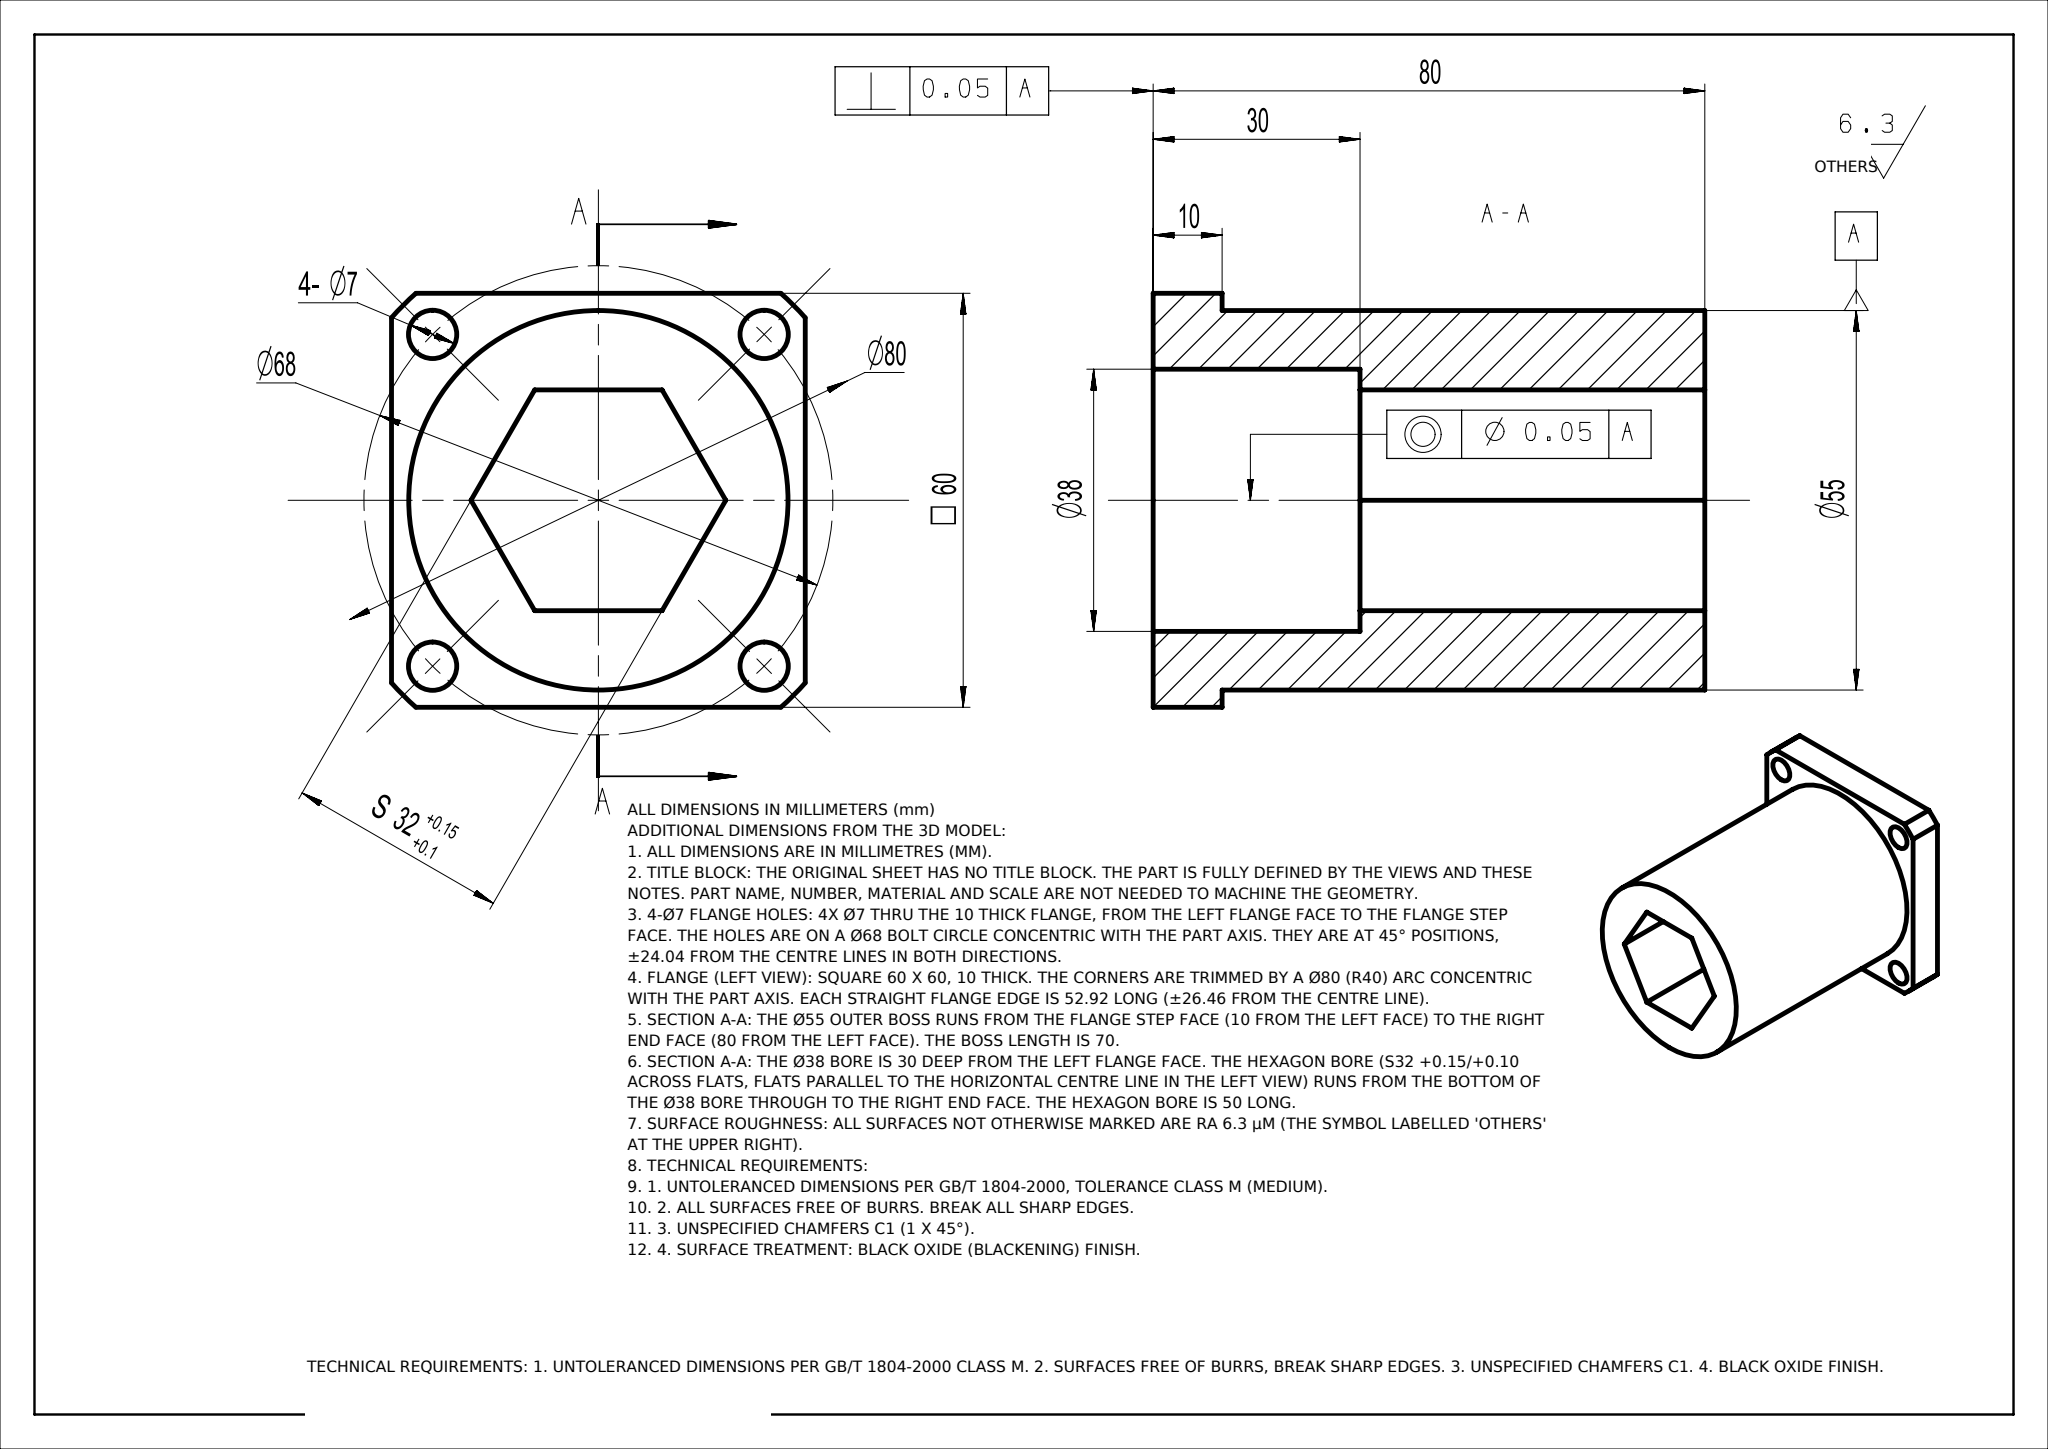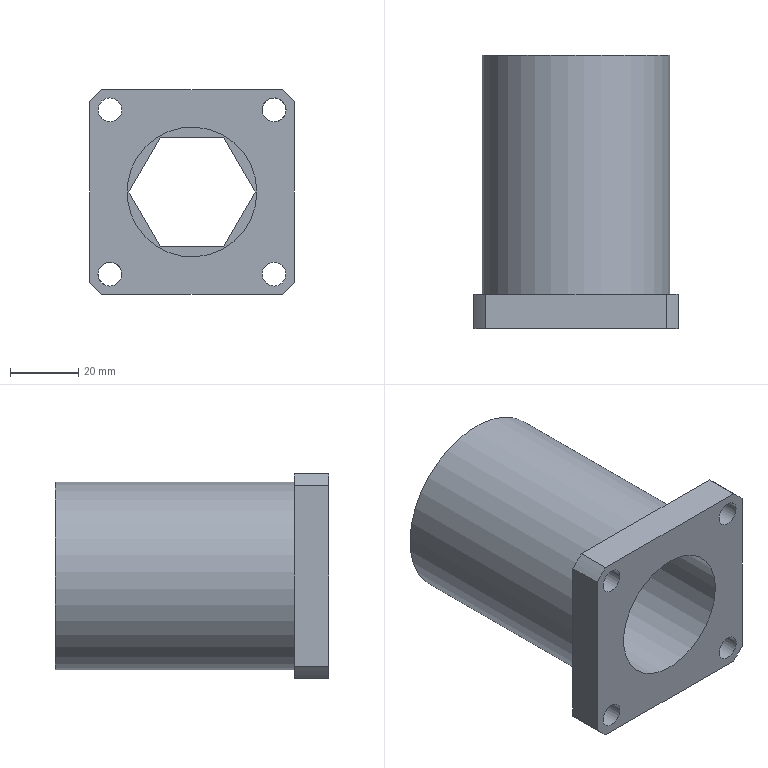Part | NX | mm | 1 solid | 24 faces | box 60 x 80 x 60 mm | volume 122164 mm3 | plane 14 | cylinder 10 | commonest cylinder face diameters 80 x4 7 x4 55 x1 38 x1
STEP:
#1=CARTESIAN_POINT('',(0.,0.,0.));
#2=DIRECTION('',(0.,0.,1.));
#3=DIRECTION('',(1.,0.,0.));
#4=AXIS2_PLACEMENT_3D('',#1,#2,#3);
#5=(LENGTH_UNIT()NAMED_UNIT(*)SI_UNIT(.MILLI.,.METRE.));
#6=UNCERTAINTY_MEASURE_WITH_UNIT(LENGTH_MEASURE(0.00002),#5,'','');
#7=(NAMED_UNIT(*)PLANE_ANGLE_UNIT()SI_UNIT($,.RADIAN.));
#8=PLANE_ANGLE_MEASURE_WITH_UNIT(PLANE_ANGLE_MEASURE(0.01745),#7);
#9=DIMENSIONAL_EXPONENTS(0.,0.,0.,0.,0.,0.,0.);
#10=(CONVERSION_BASED_UNIT('',#8)NAMED_UNIT(#9)PLANE_ANGLE_UNIT());
#11=(NAMED_UNIT(*)SI_UNIT($,.STERADIAN.)SOLID_ANGLE_UNIT());
#12=(GEOMETRIC_REPRESENTATION_CONTEXT(3)GLOBAL_UNCERTAINTY_ASSIGNED_CONTEXT((#6))GLOBAL_UNIT_ASSIGNED_CONTEXT((#5,#10,#11))REPRESENTATION_CONTEXT('',''));
#13=SHAPE_REPRESENTATION('',(#4),#12);
#14=CARTESIAN_POINT('',(-26.458,10.,30.));
#15=VERTEX_POINT('',#14);
#16=CARTESIAN_POINT('',(-30.,10.,26.458));
#17=VERTEX_POINT('',#16);
#18=CARTESIAN_POINT('',(0.,10.,0.));
#19=DIRECTION('',(0.,-1.,0.));
#20=DIRECTION('',(0.,-0.,-1.));
#21=AXIS2_PLACEMENT_3D('',#18,#19,#20);
#22=CIRCLE('',#21,40.);
#23=EDGE_CURVE('',#15,#17,#22,.T.);
#24=ORIENTED_EDGE('',*,*,#23,.T.);
#25=CARTESIAN_POINT('',(-30.,-0.,26.458));
#26=VERTEX_POINT('',#25);
#27=CARTESIAN_POINT('',(-30.,80.,26.458));
#28=DIRECTION('',(0.,-1.,0.));
#29=VECTOR('',#28,1.);
#30=LINE('',#27,#29);
#31=EDGE_CURVE('',#17,#26,#30,.T.);
#32=ORIENTED_EDGE('',*,*,#31,.T.);
#33=CARTESIAN_POINT('',(-26.458,-0.,30.));
#34=VERTEX_POINT('',#33);
#35=CARTESIAN_POINT('',(0.,-0.,0.));
#36=DIRECTION('',(0.,-1.,0.));
#37=DIRECTION('',(0.,-0.,-1.));
#38=AXIS2_PLACEMENT_3D('',#35,#36,#37);
#39=CIRCLE('',#38,40.);
#40=EDGE_CURVE('',#34,#26,#39,.T.);
#41=ORIENTED_EDGE('',*,*,#40,.F.);
#42=CARTESIAN_POINT('',(-26.458,80.,30.));
#43=DIRECTION('',(0.,1.,-0.));
#44=VECTOR('',#43,1.);
#45=LINE('',#42,#44);
#46=EDGE_CURVE('',#34,#15,#45,.T.);
#47=ORIENTED_EDGE('',*,*,#46,.T.);
#48=EDGE_LOOP('',(#24,#32,#41,#47));
#49=FACE_OUTER_BOUND('',#48,.T.);
#50=CARTESIAN_POINT('',(0.,80.,0.));
#51=DIRECTION('',(0.,-1.,0.));
#52=DIRECTION('',(0.,-0.,-1.));
#53=AXIS2_PLACEMENT_3D('',#50,#51,#52);
#54=CYLINDRICAL_SURFACE('',#53,40.);
#55=ADVANCED_FACE('',(#49),#54,.T.);
#56=CARTESIAN_POINT('',(-30.,-0.,-26.458));
#57=VERTEX_POINT('',#56);
#58=CARTESIAN_POINT('',(-26.458,-0.,-30.));
#59=VERTEX_POINT('',#58);
#60=CARTESIAN_POINT('',(0.,-0.,0.));
#61=DIRECTION('',(0.,-1.,0.));
#62=DIRECTION('',(0.,-0.,-1.));
#63=AXIS2_PLACEMENT_3D('',#60,#61,#62);
#64=CIRCLE('',#63,40.);
#65=EDGE_CURVE('',#57,#59,#64,.T.);
#66=ORIENTED_EDGE('',*,*,#65,.F.);
#67=CARTESIAN_POINT('',(-30.,10.,-26.458));
#68=VERTEX_POINT('',#67);
#69=CARTESIAN_POINT('',(-30.,80.,-26.458));
#70=DIRECTION('',(0.,1.,-0.));
#71=VECTOR('',#70,1.);
#72=LINE('',#69,#71);
#73=EDGE_CURVE('',#57,#68,#72,.T.);
#74=ORIENTED_EDGE('',*,*,#73,.T.);
#75=CARTESIAN_POINT('',(-26.458,10.,-30.));
#76=VERTEX_POINT('',#75);
#77=CARTESIAN_POINT('',(0.,10.,0.));
#78=DIRECTION('',(0.,-1.,0.));
#79=DIRECTION('',(0.,-0.,-1.));
#80=AXIS2_PLACEMENT_3D('',#77,#78,#79);
#81=CIRCLE('',#80,40.);
#82=EDGE_CURVE('',#68,#76,#81,.T.);
#83=ORIENTED_EDGE('',*,*,#82,.T.);
#84=CARTESIAN_POINT('',(-26.458,80.,-30.));
#85=DIRECTION('',(0.,-1.,0.));
#86=VECTOR('',#85,1.);
#87=LINE('',#84,#86);
#88=EDGE_CURVE('',#76,#59,#87,.T.);
#89=ORIENTED_EDGE('',*,*,#88,.T.);
#90=EDGE_LOOP('',(#66,#74,#83,#89));
#91=FACE_OUTER_BOUND('',#90,.T.);
#92=CARTESIAN_POINT('',(0.,80.,0.));
#93=DIRECTION('',(0.,-1.,0.));
#94=DIRECTION('',(0.,-0.,-1.));
#95=AXIS2_PLACEMENT_3D('',#92,#93,#94);
#96=CYLINDRICAL_SURFACE('',#95,40.);
#97=ADVANCED_FACE('',(#91),#96,.T.);
#98=CARTESIAN_POINT('',(26.458,-0.,-30.));
#99=VERTEX_POINT('',#98);
#100=CARTESIAN_POINT('',(30.,-0.,-26.458));
#101=VERTEX_POINT('',#100);
#102=CARTESIAN_POINT('',(0.,-0.,0.));
#103=DIRECTION('',(0.,-1.,0.));
#104=DIRECTION('',(0.,-0.,-1.));
#105=AXIS2_PLACEMENT_3D('',#102,#103,#104);
#106=CIRCLE('',#105,40.);
#107=EDGE_CURVE('',#99,#101,#106,.T.);
#108=ORIENTED_EDGE('',*,*,#107,.F.);
#109=CARTESIAN_POINT('',(26.458,10.,-30.));
#110=VERTEX_POINT('',#109);
#111=CARTESIAN_POINT('',(26.458,80.,-30.));
#112=DIRECTION('',(0.,1.,-0.));
#113=VECTOR('',#112,1.);
#114=LINE('',#111,#113);
#115=EDGE_CURVE('',#99,#110,#114,.T.);
#116=ORIENTED_EDGE('',*,*,#115,.T.);
#117=CARTESIAN_POINT('',(30.,10.,-26.458));
#118=VERTEX_POINT('',#117);
#119=CARTESIAN_POINT('',(0.,10.,0.));
#120=DIRECTION('',(0.,-1.,0.));
#121=DIRECTION('',(0.,-0.,-1.));
#122=AXIS2_PLACEMENT_3D('',#119,#120,#121);
#123=CIRCLE('',#122,40.);
#124=EDGE_CURVE('',#110,#118,#123,.T.);
#125=ORIENTED_EDGE('',*,*,#124,.T.);
#126=CARTESIAN_POINT('',(30.,80.,-26.458));
#127=DIRECTION('',(0.,-1.,0.));
#128=VECTOR('',#127,1.);
#129=LINE('',#126,#128);
#130=EDGE_CURVE('',#118,#101,#129,.T.);
#131=ORIENTED_EDGE('',*,*,#130,.T.);
#132=EDGE_LOOP('',(#108,#116,#125,#131));
#133=FACE_OUTER_BOUND('',#132,.T.);
#134=CARTESIAN_POINT('',(0.,80.,0.));
#135=DIRECTION('',(0.,-1.,0.));
#136=DIRECTION('',(0.,-0.,-1.));
#137=AXIS2_PLACEMENT_3D('',#134,#135,#136);
#138=CYLINDRICAL_SURFACE('',#137,40.);
#139=ADVANCED_FACE('',(#133),#138,.T.);
#140=CARTESIAN_POINT('',(-9.238,30.,-16.));
#141=VERTEX_POINT('',#140);
#142=CARTESIAN_POINT('',(-18.475,30.,0.));
#143=VERTEX_POINT('',#142);
#144=CARTESIAN_POINT('',(-18.475,30.,0.));
#145=DIRECTION('',(-0.5,0.,0.866));
#146=VECTOR('',#145,1.);
#147=LINE('',#144,#146);
#148=EDGE_CURVE('',#141,#143,#147,.T.);
#149=ORIENTED_EDGE('',*,*,#148,.F.);
#150=CARTESIAN_POINT('',(-9.238,80.,-16.));
#151=VERTEX_POINT('',#150);
#152=CARTESIAN_POINT('',(-9.238,100.,-16.));
#153=DIRECTION('',(0.,1.,0.));
#154=VECTOR('',#153,1.);
#155=LINE('',#152,#154);
#156=EDGE_CURVE('',#141,#151,#155,.T.);
#157=ORIENTED_EDGE('',*,*,#156,.T.);
#158=CARTESIAN_POINT('',(-18.475,80.,0.));
#159=VERTEX_POINT('',#158);
#160=CARTESIAN_POINT('',(-13.856,80.,-8.));
#161=DIRECTION('',(0.5,-0.,-0.866));
#162=VECTOR('',#161,1.);
#163=LINE('',#160,#162);
#164=EDGE_CURVE('',#159,#151,#163,.T.);
#165=ORIENTED_EDGE('',*,*,#164,.F.);
#166=CARTESIAN_POINT('',(-18.475,100.,0.));
#167=DIRECTION('',(0.,1.,0.));
#168=VECTOR('',#167,1.);
#169=LINE('',#166,#168);
#170=EDGE_CURVE('',#143,#159,#169,.T.);
#171=ORIENTED_EDGE('',*,*,#170,.F.);
#172=EDGE_LOOP('',(#149,#157,#165,#171));
#173=FACE_OUTER_BOUND('',#172,.T.);
#174=CARTESIAN_POINT('',(-18.475,100.,0.));
#175=DIRECTION('',(-0.866,0.,-0.5));
#176=DIRECTION('',(-0.5,0.,0.866));
#177=AXIS2_PLACEMENT_3D('',#174,#175,#176);
#178=PLANE('',#177);
#179=ADVANCED_FACE('',(#173),#178,.F.);
#180=CARTESIAN_POINT('',(9.238,30.,-16.));
#181=VERTEX_POINT('',#180);
#182=CARTESIAN_POINT('',(-9.238,30.,-16.));
#183=DIRECTION('',(-1.,0.,0.));
#184=VECTOR('',#183,1.);
#185=LINE('',#182,#184);
#186=EDGE_CURVE('',#181,#141,#185,.T.);
#187=ORIENTED_EDGE('',*,*,#186,.F.);
#188=CARTESIAN_POINT('',(9.238,80.,-16.));
#189=VERTEX_POINT('',#188);
#190=CARTESIAN_POINT('',(9.238,100.,-16.));
#191=DIRECTION('',(0.,1.,0.));
#192=VECTOR('',#191,1.);
#193=LINE('',#190,#192);
#194=EDGE_CURVE('',#181,#189,#193,.T.);
#195=ORIENTED_EDGE('',*,*,#194,.T.);
#196=CARTESIAN_POINT('',(-0.,80.,-16.));
#197=DIRECTION('',(1.,-0.,-0.));
#198=VECTOR('',#197,1.);
#199=LINE('',#196,#198);
#200=EDGE_CURVE('',#151,#189,#199,.T.);
#201=ORIENTED_EDGE('',*,*,#200,.F.);
#202=ORIENTED_EDGE('',*,*,#156,.F.);
#203=EDGE_LOOP('',(#187,#195,#201,#202));
#204=FACE_OUTER_BOUND('',#203,.T.);
#205=CARTESIAN_POINT('',(-9.238,100.,-16.));
#206=DIRECTION('',(-0.,0.,-1.));
#207=DIRECTION('',(-1.,0.,0.));
#208=AXIS2_PLACEMENT_3D('',#205,#206,#207);
#209=PLANE('',#208);
#210=ADVANCED_FACE('',(#204),#209,.F.);
#211=CARTESIAN_POINT('',(18.475,30.,0.));
#212=VERTEX_POINT('',#211);
#213=CARTESIAN_POINT('',(9.238,30.,-16.));
#214=DIRECTION('',(-0.5,0.,-0.866));
#215=VECTOR('',#214,1.);
#216=LINE('',#213,#215);
#217=EDGE_CURVE('',#212,#181,#216,.T.);
#218=ORIENTED_EDGE('',*,*,#217,.F.);
#219=CARTESIAN_POINT('',(18.475,80.,0.));
#220=VERTEX_POINT('',#219);
#221=CARTESIAN_POINT('',(18.475,100.,0.));
#222=DIRECTION('',(0.,1.,0.));
#223=VECTOR('',#222,1.);
#224=LINE('',#221,#223);
#225=EDGE_CURVE('',#212,#220,#224,.T.);
#226=ORIENTED_EDGE('',*,*,#225,.T.);
#227=CARTESIAN_POINT('',(13.856,80.,-8.));
#228=DIRECTION('',(0.5,0.,0.866));
#229=VECTOR('',#228,1.);
#230=LINE('',#227,#229);
#231=EDGE_CURVE('',#189,#220,#230,.T.);
#232=ORIENTED_EDGE('',*,*,#231,.F.);
#233=ORIENTED_EDGE('',*,*,#194,.F.);
#234=EDGE_LOOP('',(#218,#226,#232,#233));
#235=FACE_OUTER_BOUND('',#234,.T.);
#236=CARTESIAN_POINT('',(9.238,100.,-16.));
#237=DIRECTION('',(0.866,0.,-0.5));
#238=DIRECTION('',(-0.5,0.,-0.866));
#239=AXIS2_PLACEMENT_3D('',#236,#237,#238);
#240=PLANE('',#239);
#241=ADVANCED_FACE('',(#235),#240,.F.);
#242=CARTESIAN_POINT('',(9.238,30.,16.));
#243=VERTEX_POINT('',#242);
#244=CARTESIAN_POINT('',(18.475,30.,0.));
#245=DIRECTION('',(0.5,0.,-0.866));
#246=VECTOR('',#245,1.);
#247=LINE('',#244,#246);
#248=EDGE_CURVE('',#243,#212,#247,.T.);
#249=ORIENTED_EDGE('',*,*,#248,.F.);
#250=CARTESIAN_POINT('',(9.238,80.,16.));
#251=VERTEX_POINT('',#250);
#252=CARTESIAN_POINT('',(9.238,100.,16.));
#253=DIRECTION('',(0.,1.,0.));
#254=VECTOR('',#253,1.);
#255=LINE('',#252,#254);
#256=EDGE_CURVE('',#243,#251,#255,.T.);
#257=ORIENTED_EDGE('',*,*,#256,.T.);
#258=CARTESIAN_POINT('',(13.856,80.,8.));
#259=DIRECTION('',(-0.5,0.,0.866));
#260=VECTOR('',#259,1.);
#261=LINE('',#258,#260);
#262=EDGE_CURVE('',#220,#251,#261,.T.);
#263=ORIENTED_EDGE('',*,*,#262,.F.);
#264=ORIENTED_EDGE('',*,*,#225,.F.);
#265=EDGE_LOOP('',(#249,#257,#263,#264));
#266=FACE_OUTER_BOUND('',#265,.T.);
#267=CARTESIAN_POINT('',(18.475,100.,0.));
#268=DIRECTION('',(0.866,0.,0.5));
#269=DIRECTION('',(0.5,0.,-0.866));
#270=AXIS2_PLACEMENT_3D('',#267,#268,#269);
#271=PLANE('',#270);
#272=ADVANCED_FACE('',(#266),#271,.F.);
#273=CARTESIAN_POINT('',(-9.238,30.,16.));
#274=VERTEX_POINT('',#273);
#275=CARTESIAN_POINT('',(9.238,30.,16.));
#276=DIRECTION('',(1.,0.,-0.));
#277=VECTOR('',#276,1.);
#278=LINE('',#275,#277);
#279=EDGE_CURVE('',#274,#243,#278,.T.);
#280=ORIENTED_EDGE('',*,*,#279,.F.);
#281=CARTESIAN_POINT('',(-9.238,80.,16.));
#282=VERTEX_POINT('',#281);
#283=CARTESIAN_POINT('',(-9.238,100.,16.));
#284=DIRECTION('',(0.,1.,0.));
#285=VECTOR('',#284,1.);
#286=LINE('',#283,#285);
#287=EDGE_CURVE('',#274,#282,#286,.T.);
#288=ORIENTED_EDGE('',*,*,#287,.T.);
#289=CARTESIAN_POINT('',(0.,80.,16.));
#290=DIRECTION('',(-1.,0.,0.));
#291=VECTOR('',#290,1.);
#292=LINE('',#289,#291);
#293=EDGE_CURVE('',#251,#282,#292,.T.);
#294=ORIENTED_EDGE('',*,*,#293,.F.);
#295=ORIENTED_EDGE('',*,*,#256,.F.);
#296=EDGE_LOOP('',(#280,#288,#294,#295));
#297=FACE_OUTER_BOUND('',#296,.T.);
#298=CARTESIAN_POINT('',(9.238,100.,16.));
#299=DIRECTION('',(0.,0.,1.));
#300=DIRECTION('',(1.,0.,-0.));
#301=AXIS2_PLACEMENT_3D('',#298,#299,#300);
#302=PLANE('',#301);
#303=ADVANCED_FACE('',(#297),#302,.F.);
#304=CARTESIAN_POINT('',(-9.238,30.,16.));
#305=DIRECTION('',(0.5,0.,0.866));
#306=VECTOR('',#305,1.);
#307=LINE('',#304,#306);
#308=EDGE_CURVE('',#143,#274,#307,.T.);
#309=ORIENTED_EDGE('',*,*,#308,.F.);
#310=ORIENTED_EDGE('',*,*,#170,.T.);
#311=CARTESIAN_POINT('',(-13.856,80.,8.));
#312=DIRECTION('',(-0.5,-0.,-0.866));
#313=VECTOR('',#312,1.);
#314=LINE('',#311,#313);
#315=EDGE_CURVE('',#282,#159,#314,.T.);
#316=ORIENTED_EDGE('',*,*,#315,.F.);
#317=ORIENTED_EDGE('',*,*,#287,.F.);
#318=EDGE_LOOP('',(#309,#310,#316,#317));
#319=FACE_OUTER_BOUND('',#318,.T.);
#320=CARTESIAN_POINT('',(-9.238,100.,16.));
#321=DIRECTION('',(-0.866,0.,0.5));
#322=DIRECTION('',(0.5,0.,0.866));
#323=AXIS2_PLACEMENT_3D('',#320,#321,#322);
#324=PLANE('',#323);
#325=ADVANCED_FACE('',(#319),#324,.F.);
#326=CARTESIAN_POINT('',(19.,-0.,-0.));
#327=VERTEX_POINT('',#326);
#328=CARTESIAN_POINT('',(0.,-0.,0.));
#329=DIRECTION('',(0.,-1.,0.));
#330=DIRECTION('',(1.,0.,-0.));
#331=AXIS2_PLACEMENT_3D('',#328,#329,#330);
#332=CIRCLE('',#331,19.);
#333=EDGE_CURVE('',#327,#327,#332,.T.);
#334=ORIENTED_EDGE('',*,*,#333,.F.);
#335=EDGE_LOOP('',(#334));
#336=FACE_BOUND('',#335,.T.);
#337=CARTESIAN_POINT('',(27.542,-0.,24.042));
#338=VERTEX_POINT('',#337);
#339=CARTESIAN_POINT('',(24.042,-0.,24.042));
#340=DIRECTION('',(0.,-1.,0.));
#341=DIRECTION('',(1.,0.,0.));
#342=AXIS2_PLACEMENT_3D('',#339,#340,#341);
#343=CIRCLE('',#342,3.5);
#344=EDGE_CURVE('',#338,#338,#343,.T.);
#345=ORIENTED_EDGE('',*,*,#344,.F.);
#346=EDGE_LOOP('',(#345));
#347=FACE_BOUND('',#346,.T.);
#348=CARTESIAN_POINT('',(-24.042,0.,27.542));
#349=VERTEX_POINT('',#348);
#350=CARTESIAN_POINT('',(-24.042,0.,24.042));
#351=DIRECTION('',(0.,-1.,0.));
#352=DIRECTION('',(0.,0.,1.));
#353=AXIS2_PLACEMENT_3D('',#350,#351,#352);
#354=CIRCLE('',#353,3.5);
#355=EDGE_CURVE('',#349,#349,#354,.T.);
#356=ORIENTED_EDGE('',*,*,#355,.F.);
#357=EDGE_LOOP('',(#356));
#358=FACE_BOUND('',#357,.T.);
#359=CARTESIAN_POINT('',(-27.542,-0.,-24.042));
#360=VERTEX_POINT('',#359);
#361=CARTESIAN_POINT('',(-24.042,-0.,-24.042));
#362=DIRECTION('',(0.,-1.,0.));
#363=DIRECTION('',(-1.,0.,0.));
#364=AXIS2_PLACEMENT_3D('',#361,#362,#363);
#365=CIRCLE('',#364,3.5);
#366=EDGE_CURVE('',#360,#360,#365,.T.);
#367=ORIENTED_EDGE('',*,*,#366,.F.);
#368=EDGE_LOOP('',(#367));
#369=FACE_BOUND('',#368,.T.);
#370=CARTESIAN_POINT('',(24.042,-0.,-27.542));
#371=VERTEX_POINT('',#370);
#372=CARTESIAN_POINT('',(24.042,-0.,-24.042));
#373=DIRECTION('',(0.,-1.,0.));
#374=DIRECTION('',(0.,-0.,-1.));
#375=AXIS2_PLACEMENT_3D('',#372,#373,#374);
#376=CIRCLE('',#375,3.5);
#377=EDGE_CURVE('',#371,#371,#376,.T.);
#378=ORIENTED_EDGE('',*,*,#377,.F.);
#379=EDGE_LOOP('',(#378));
#380=FACE_BOUND('',#379,.T.);
#381=CARTESIAN_POINT('',(30.,-0.,26.458));
#382=VERTEX_POINT('',#381);
#383=CARTESIAN_POINT('',(26.458,-0.,30.));
#384=VERTEX_POINT('',#383);
#385=CARTESIAN_POINT('',(0.,-0.,0.));
#386=DIRECTION('',(0.,-1.,0.));
#387=DIRECTION('',(0.,-0.,-1.));
#388=AXIS2_PLACEMENT_3D('',#385,#386,#387);
#389=CIRCLE('',#388,40.);
#390=EDGE_CURVE('',#382,#384,#389,.T.);
#391=ORIENTED_EDGE('',*,*,#390,.T.);
#392=CARTESIAN_POINT('',(30.,-0.,30.));
#393=DIRECTION('',(-1.,0.,-0.));
#394=VECTOR('',#393,1.);
#395=LINE('',#392,#394);
#396=EDGE_CURVE('',#384,#34,#395,.T.);
#397=ORIENTED_EDGE('',*,*,#396,.T.);
#398=ORIENTED_EDGE('',*,*,#40,.T.);
#399=CARTESIAN_POINT('',(-30.,-0.,30.));
#400=DIRECTION('',(0.,0.,-1.));
#401=VECTOR('',#400,1.);
#402=LINE('',#399,#401);
#403=EDGE_CURVE('',#26,#57,#402,.T.);
#404=ORIENTED_EDGE('',*,*,#403,.T.);
#405=ORIENTED_EDGE('',*,*,#65,.T.);
#406=CARTESIAN_POINT('',(-30.,-0.,-30.));
#407=DIRECTION('',(1.,0.,-0.));
#408=VECTOR('',#407,1.);
#409=LINE('',#406,#408);
#410=EDGE_CURVE('',#59,#99,#409,.T.);
#411=ORIENTED_EDGE('',*,*,#410,.T.);
#412=ORIENTED_EDGE('',*,*,#107,.T.);
#413=CARTESIAN_POINT('',(30.,-0.,-30.));
#414=DIRECTION('',(0.,0.,1.));
#415=VECTOR('',#414,1.);
#416=LINE('',#413,#415);
#417=EDGE_CURVE('',#101,#382,#416,.T.);
#418=ORIENTED_EDGE('',*,*,#417,.T.);
#419=EDGE_LOOP('',(#391,#397,#398,#404,#405,#411,#412,#418));
#420=FACE_BOUND('',#419,.T.);
#421=CARTESIAN_POINT('',(0.,0.,40.));
#422=DIRECTION('',(0.,1.,-0.));
#423=DIRECTION('',(0.,0.,1.));
#424=AXIS2_PLACEMENT_3D('',#421,#422,#423);
#425=PLANE('',#424);
#426=ADVANCED_FACE('',(#336,#347,#358,#369,#380,#420),#425,.F.);
#427=ORIENTED_EDGE('',*,*,#315,.T.);
#428=ORIENTED_EDGE('',*,*,#164,.T.);
#429=ORIENTED_EDGE('',*,*,#200,.T.);
#430=ORIENTED_EDGE('',*,*,#231,.T.);
#431=ORIENTED_EDGE('',*,*,#262,.T.);
#432=ORIENTED_EDGE('',*,*,#293,.T.);
#433=EDGE_LOOP('',(#427,#428,#429,#430,#431,#432));
#434=FACE_BOUND('',#433,.T.);
#435=CARTESIAN_POINT('',(0.,80.,-27.5));
#436=VERTEX_POINT('',#435);
#437=CARTESIAN_POINT('',(0.,80.,0.));
#438=DIRECTION('',(0.,-1.,0.));
#439=DIRECTION('',(0.,-0.,-1.));
#440=AXIS2_PLACEMENT_3D('',#437,#438,#439);
#441=CIRCLE('',#440,27.5);
#442=EDGE_CURVE('',#436,#436,#441,.T.);
#443=ORIENTED_EDGE('',*,*,#442,.F.);
#444=EDGE_LOOP('',(#443));
#445=FACE_BOUND('',#444,.T.);
#446=CARTESIAN_POINT('',(0.,80.,0.));
#447=DIRECTION('',(0.,-1.,0.));
#448=DIRECTION('',(0.,-0.,-1.));
#449=AXIS2_PLACEMENT_3D('',#446,#447,#448);
#450=PLANE('',#449);
#451=ADVANCED_FACE('',(#434,#445),#450,.F.);
#452=CARTESIAN_POINT('',(0.,10.,-27.5));
#453=VERTEX_POINT('',#452);
#454=CARTESIAN_POINT('',(0.,10.,0.));
#455=DIRECTION('',(0.,-1.,0.));
#456=DIRECTION('',(0.,-0.,-1.));
#457=AXIS2_PLACEMENT_3D('',#454,#455,#456);
#458=CIRCLE('',#457,27.5);
#459=EDGE_CURVE('',#453,#453,#458,.T.);
#460=ORIENTED_EDGE('',*,*,#459,.F.);
#461=EDGE_LOOP('',(#460));
#462=FACE_BOUND('',#461,.T.);
#463=ORIENTED_EDGE('',*,*,#442,.T.);
#464=EDGE_LOOP('',(#463));
#465=FACE_BOUND('',#464,.T.);
#466=CARTESIAN_POINT('',(0.,80.,0.));
#467=DIRECTION('',(0.,-1.,0.));
#468=DIRECTION('',(0.,-0.,-1.));
#469=AXIS2_PLACEMENT_3D('',#466,#467,#468);
#470=CYLINDRICAL_SURFACE('',#469,27.5);
#471=ADVANCED_FACE('',(#462,#465),#470,.T.);
#472=CARTESIAN_POINT('',(24.042,10.,20.542));
#473=VERTEX_POINT('',#472);
#474=CARTESIAN_POINT('',(24.042,10.,24.042));
#475=DIRECTION('',(0.,-1.,0.));
#476=DIRECTION('',(0.,-0.,-1.));
#477=AXIS2_PLACEMENT_3D('',#474,#475,#476);
#478=CIRCLE('',#477,3.5);
#479=EDGE_CURVE('',#473,#473,#478,.T.);
#480=ORIENTED_EDGE('',*,*,#479,.T.);
#481=EDGE_LOOP('',(#480));
#482=FACE_BOUND('',#481,.T.);
#483=CARTESIAN_POINT('',(-24.042,10.,20.542));
#484=VERTEX_POINT('',#483);
#485=CARTESIAN_POINT('',(-24.042,10.,24.042));
#486=DIRECTION('',(0.,-1.,0.));
#487=DIRECTION('',(0.,-0.,-1.));
#488=AXIS2_PLACEMENT_3D('',#485,#486,#487);
#489=CIRCLE('',#488,3.5);
#490=EDGE_CURVE('',#484,#484,#489,.T.);
#491=ORIENTED_EDGE('',*,*,#490,.T.);
#492=EDGE_LOOP('',(#491));
#493=FACE_BOUND('',#492,.T.);
#494=CARTESIAN_POINT('',(-24.042,10.,-27.542));
#495=VERTEX_POINT('',#494);
#496=CARTESIAN_POINT('',(-24.042,10.,-24.042));
#497=DIRECTION('',(0.,-1.,0.));
#498=DIRECTION('',(0.,-0.,-1.));
#499=AXIS2_PLACEMENT_3D('',#496,#497,#498);
#500=CIRCLE('',#499,3.5);
#501=EDGE_CURVE('',#495,#495,#500,.T.);
#502=ORIENTED_EDGE('',*,*,#501,.T.);
#503=EDGE_LOOP('',(#502));
#504=FACE_BOUND('',#503,.T.);
#505=CARTESIAN_POINT('',(24.042,10.,-27.542));
#506=VERTEX_POINT('',#505);
#507=CARTESIAN_POINT('',(24.042,10.,-24.042));
#508=DIRECTION('',(0.,-1.,0.));
#509=DIRECTION('',(0.,-0.,-1.));
#510=AXIS2_PLACEMENT_3D('',#507,#508,#509);
#511=CIRCLE('',#510,3.5);
#512=EDGE_CURVE('',#506,#506,#511,.T.);
#513=ORIENTED_EDGE('',*,*,#512,.T.);
#514=EDGE_LOOP('',(#513));
#515=FACE_BOUND('',#514,.T.);
#516=ORIENTED_EDGE('',*,*,#82,.F.);
#517=CARTESIAN_POINT('',(-30.,10.,27.5));
#518=DIRECTION('',(0.,0.,1.));
#519=VECTOR('',#518,1.);
#520=LINE('',#517,#519);
#521=EDGE_CURVE('',#68,#17,#520,.T.);
#522=ORIENTED_EDGE('',*,*,#521,.T.);
#523=ORIENTED_EDGE('',*,*,#23,.F.);
#524=CARTESIAN_POINT('',(26.458,10.,30.));
#525=VERTEX_POINT('',#524);
#526=CARTESIAN_POINT('',(-0.,10.,30.));
#527=DIRECTION('',(1.,0.,0.));
#528=VECTOR('',#527,1.);
#529=LINE('',#526,#528);
#530=EDGE_CURVE('',#15,#525,#529,.T.);
#531=ORIENTED_EDGE('',*,*,#530,.T.);
#532=CARTESIAN_POINT('',(30.,10.,26.458));
#533=VERTEX_POINT('',#532);
#534=CARTESIAN_POINT('',(0.,10.,0.));
#535=DIRECTION('',(0.,-1.,0.));
#536=DIRECTION('',(0.,-0.,-1.));
#537=AXIS2_PLACEMENT_3D('',#534,#535,#536);
#538=CIRCLE('',#537,40.);
#539=EDGE_CURVE('',#533,#525,#538,.T.);
#540=ORIENTED_EDGE('',*,*,#539,.F.);
#541=CARTESIAN_POINT('',(30.,10.,27.5));
#542=DIRECTION('',(0.,-0.,-1.));
#543=VECTOR('',#542,1.);
#544=LINE('',#541,#543);
#545=EDGE_CURVE('',#533,#118,#544,.T.);
#546=ORIENTED_EDGE('',*,*,#545,.T.);
#547=ORIENTED_EDGE('',*,*,#124,.F.);
#548=CARTESIAN_POINT('',(-0.,10.,-30.));
#549=DIRECTION('',(-1.,0.,0.));
#550=VECTOR('',#549,1.);
#551=LINE('',#548,#550);
#552=EDGE_CURVE('',#110,#76,#551,.T.);
#553=ORIENTED_EDGE('',*,*,#552,.T.);
#554=EDGE_LOOP('',(#516,#522,#523,#531,#540,#546,#547,#553));
#555=FACE_BOUND('',#554,.T.);
#556=ORIENTED_EDGE('',*,*,#459,.T.);
#557=EDGE_LOOP('',(#556));
#558=FACE_BOUND('',#557,.T.);
#559=CARTESIAN_POINT('',(0.,10.,27.5));
#560=DIRECTION('',(0.,-1.,0.));
#561=DIRECTION('',(0.,-0.,-1.));
#562=AXIS2_PLACEMENT_3D('',#559,#560,#561);
#563=PLANE('',#562);
#564=ADVANCED_FACE('',(#482,#493,#504,#515,#555,#558),#563,.F.);
#565=ORIENTED_EDGE('',*,*,#390,.F.);
#566=CARTESIAN_POINT('',(30.,80.,26.458));
#567=DIRECTION('',(0.,1.,-0.));
#568=VECTOR('',#567,1.);
#569=LINE('',#566,#568);
#570=EDGE_CURVE('',#382,#533,#569,.T.);
#571=ORIENTED_EDGE('',*,*,#570,.T.);
#572=ORIENTED_EDGE('',*,*,#539,.T.);
#573=CARTESIAN_POINT('',(26.458,80.,30.));
#574=DIRECTION('',(0.,-1.,0.));
#575=VECTOR('',#574,1.);
#576=LINE('',#573,#575);
#577=EDGE_CURVE('',#525,#384,#576,.T.);
#578=ORIENTED_EDGE('',*,*,#577,.T.);
#579=EDGE_LOOP('',(#565,#571,#572,#578));
#580=FACE_OUTER_BOUND('',#579,.T.);
#581=CARTESIAN_POINT('',(0.,80.,0.));
#582=DIRECTION('',(0.,-1.,0.));
#583=DIRECTION('',(0.,-0.,-1.));
#584=AXIS2_PLACEMENT_3D('',#581,#582,#583);
#585=CYLINDRICAL_SURFACE('',#584,40.);
#586=ADVANCED_FACE('',(#580),#585,.T.);
#587=ORIENTED_EDGE('',*,*,#377,.T.);
#588=EDGE_LOOP('',(#587));
#589=FACE_BOUND('',#588,.T.);
#590=ORIENTED_EDGE('',*,*,#512,.F.);
#591=EDGE_LOOP('',(#590));
#592=FACE_BOUND('',#591,.T.);
#593=CARTESIAN_POINT('',(24.042,12.,-24.042));
#594=DIRECTION('',(0.,-1.,0.));
#595=DIRECTION('',(0.,-0.,-1.));
#596=AXIS2_PLACEMENT_3D('',#593,#594,#595);
#597=CYLINDRICAL_SURFACE('',#596,3.5);
#598=ADVANCED_FACE('',(#589,#592),#597,.F.);
#599=ORIENTED_EDGE('',*,*,#366,.T.);
#600=EDGE_LOOP('',(#599));
#601=FACE_BOUND('',#600,.T.);
#602=ORIENTED_EDGE('',*,*,#501,.F.);
#603=EDGE_LOOP('',(#602));
#604=FACE_BOUND('',#603,.T.);
#605=CARTESIAN_POINT('',(-24.042,12.,-24.042));
#606=DIRECTION('',(0.,-1.,0.));
#607=DIRECTION('',(0.,-0.,-1.));
#608=AXIS2_PLACEMENT_3D('',#605,#606,#607);
#609=CYLINDRICAL_SURFACE('',#608,3.5);
#610=ADVANCED_FACE('',(#601,#604),#609,.F.);
#611=ORIENTED_EDGE('',*,*,#355,.T.);
#612=EDGE_LOOP('',(#611));
#613=FACE_BOUND('',#612,.T.);
#614=ORIENTED_EDGE('',*,*,#490,.F.);
#615=EDGE_LOOP('',(#614));
#616=FACE_BOUND('',#615,.T.);
#617=CARTESIAN_POINT('',(-24.042,12.,24.042));
#618=DIRECTION('',(0.,-1.,0.));
#619=DIRECTION('',(0.,-0.,-1.));
#620=AXIS2_PLACEMENT_3D('',#617,#618,#619);
#621=CYLINDRICAL_SURFACE('',#620,3.5);
#622=ADVANCED_FACE('',(#613,#616),#621,.F.);
#623=ORIENTED_EDGE('',*,*,#344,.T.);
#624=EDGE_LOOP('',(#623));
#625=FACE_BOUND('',#624,.T.);
#626=ORIENTED_EDGE('',*,*,#479,.F.);
#627=EDGE_LOOP('',(#626));
#628=FACE_BOUND('',#627,.T.);
#629=CARTESIAN_POINT('',(24.042,12.,24.042));
#630=DIRECTION('',(0.,-1.,0.));
#631=DIRECTION('',(0.,-0.,-1.));
#632=AXIS2_PLACEMENT_3D('',#629,#630,#631);
#633=CYLINDRICAL_SURFACE('',#632,3.5);
#634=ADVANCED_FACE('',(#625,#628),#633,.F.);
#635=CARTESIAN_POINT('',(19.,30.,-0.));
#636=VERTEX_POINT('',#635);
#637=CARTESIAN_POINT('',(0.,30.,0.));
#638=DIRECTION('',(0.,1.,0.));
#639=DIRECTION('',(1.,0.,-0.));
#640=AXIS2_PLACEMENT_3D('',#637,#638,#639);
#641=CIRCLE('',#640,19.);
#642=EDGE_CURVE('',#636,#636,#641,.T.);
#643=ORIENTED_EDGE('',*,*,#642,.F.);
#644=EDGE_LOOP('',(#643));
#645=FACE_BOUND('',#644,.T.);
#646=ORIENTED_EDGE('',*,*,#148,.T.);
#647=ORIENTED_EDGE('',*,*,#308,.T.);
#648=ORIENTED_EDGE('',*,*,#279,.T.);
#649=ORIENTED_EDGE('',*,*,#248,.T.);
#650=ORIENTED_EDGE('',*,*,#217,.T.);
#651=ORIENTED_EDGE('',*,*,#186,.T.);
#652=EDGE_LOOP('',(#646,#647,#648,#649,#650,#651));
#653=FACE_BOUND('',#652,.T.);
#654=CARTESIAN_POINT('',(0.,30.,0.));
#655=DIRECTION('',(0.,-1.,0.));
#656=DIRECTION('',(0.,0.,-1.));
#657=AXIS2_PLACEMENT_3D('',#654,#655,#656);
#658=PLANE('',#657);
#659=ADVANCED_FACE('',(#645,#653),#658,.T.);
#660=ORIENTED_EDGE('',*,*,#642,.T.);
#661=EDGE_LOOP('',(#660));
#662=FACE_BOUND('',#661,.T.);
#663=ORIENTED_EDGE('',*,*,#333,.T.);
#664=EDGE_LOOP('',(#663));
#665=FACE_BOUND('',#664,.T.);
#666=CARTESIAN_POINT('',(0.,30.,0.));
#667=DIRECTION('',(0.,-1.,0.));
#668=DIRECTION('',(0.,0.,-1.));
#669=AXIS2_PLACEMENT_3D('',#666,#667,#668);
#670=CYLINDRICAL_SURFACE('',#669,19.);
#671=ADVANCED_FACE('',(#662,#665),#670,.F.);
#672=ORIENTED_EDGE('',*,*,#530,.F.);
#673=ORIENTED_EDGE('',*,*,#46,.F.);
#674=ORIENTED_EDGE('',*,*,#396,.F.);
#675=ORIENTED_EDGE('',*,*,#577,.F.);
#676=EDGE_LOOP('',(#672,#673,#674,#675));
#677=FACE_OUTER_BOUND('',#676,.T.);
#678=CARTESIAN_POINT('',(30.,-0.,30.));
#679=DIRECTION('',(0.,0.,-1.));
#680=DIRECTION('',(-1.,0.,-0.));
#681=AXIS2_PLACEMENT_3D('',#678,#679,#680);
#682=PLANE('',#681);
#683=ADVANCED_FACE('',(#677),#682,.F.);
#684=ORIENTED_EDGE('',*,*,#545,.F.);
#685=ORIENTED_EDGE('',*,*,#570,.F.);
#686=ORIENTED_EDGE('',*,*,#417,.F.);
#687=ORIENTED_EDGE('',*,*,#130,.F.);
#688=EDGE_LOOP('',(#684,#685,#686,#687));
#689=FACE_OUTER_BOUND('',#688,.T.);
#690=CARTESIAN_POINT('',(30.,-0.,-30.));
#691=DIRECTION('',(-1.,0.,0.));
#692=DIRECTION('',(0.,0.,1.));
#693=AXIS2_PLACEMENT_3D('',#690,#691,#692);
#694=PLANE('',#693);
#695=ADVANCED_FACE('',(#689),#694,.F.);
#696=ORIENTED_EDGE('',*,*,#552,.F.);
#697=ORIENTED_EDGE('',*,*,#115,.F.);
#698=ORIENTED_EDGE('',*,*,#410,.F.);
#699=ORIENTED_EDGE('',*,*,#88,.F.);
#700=EDGE_LOOP('',(#696,#697,#698,#699));
#701=FACE_OUTER_BOUND('',#700,.T.);
#702=CARTESIAN_POINT('',(-30.,-0.,-30.));
#703=DIRECTION('',(0.,0.,1.));
#704=DIRECTION('',(1.,0.,-0.));
#705=AXIS2_PLACEMENT_3D('',#702,#703,#704);
#706=PLANE('',#705);
#707=ADVANCED_FACE('',(#701),#706,.F.);
#708=ORIENTED_EDGE('',*,*,#521,.F.);
#709=ORIENTED_EDGE('',*,*,#73,.F.);
#710=ORIENTED_EDGE('',*,*,#403,.F.);
#711=ORIENTED_EDGE('',*,*,#31,.F.);
#712=EDGE_LOOP('',(#708,#709,#710,#711));
#713=FACE_OUTER_BOUND('',#712,.T.);
#714=CARTESIAN_POINT('',(-30.,-0.,30.));
#715=DIRECTION('',(1.,0.,0.));
#716=DIRECTION('',(0.,0.,-1.));
#717=AXIS2_PLACEMENT_3D('',#714,#715,#716);
#718=PLANE('',#717);
#719=ADVANCED_FACE('',(#713),#718,.F.);
#720=CLOSED_SHELL('',(#55,#97,#139,#179,#210,#241,#272,#303,#325,#426,#451,#471,#564,#586,#598,#610,#622,#634,#659,#671,#683,#695,#707,#719));
#721=MANIFOLD_SOLID_BREP('',#720);
#722=ADVANCED_BREP_SHAPE_REPRESENTATION('',(#721),#12);
#723=SHAPE_REPRESENTATION_RELATIONSHIP('','',#13,#722);
#724=PRESENTATION_LAYER_ASSIGNMENT('','',(#721));
#725=COLOUR_RGB('',0.4,0.4,0.4);
#726=FILL_AREA_STYLE_COLOUR('',#725);
#727=FILL_AREA_STYLE('',(#726));
#728=SURFACE_STYLE_FILL_AREA(#727);
#729=SURFACE_SIDE_STYLE('',(#728));
#730=SURFACE_STYLE_USAGE(.BOTH.,#729);
#731=PRESENTATION_STYLE_ASSIGNMENT((#730));
#732=STYLED_ITEM('',(#731),#721);
#733=MECHANICAL_DESIGN_GEOMETRIC_PRESENTATION_REPRESENTATION('',(#732),#12);